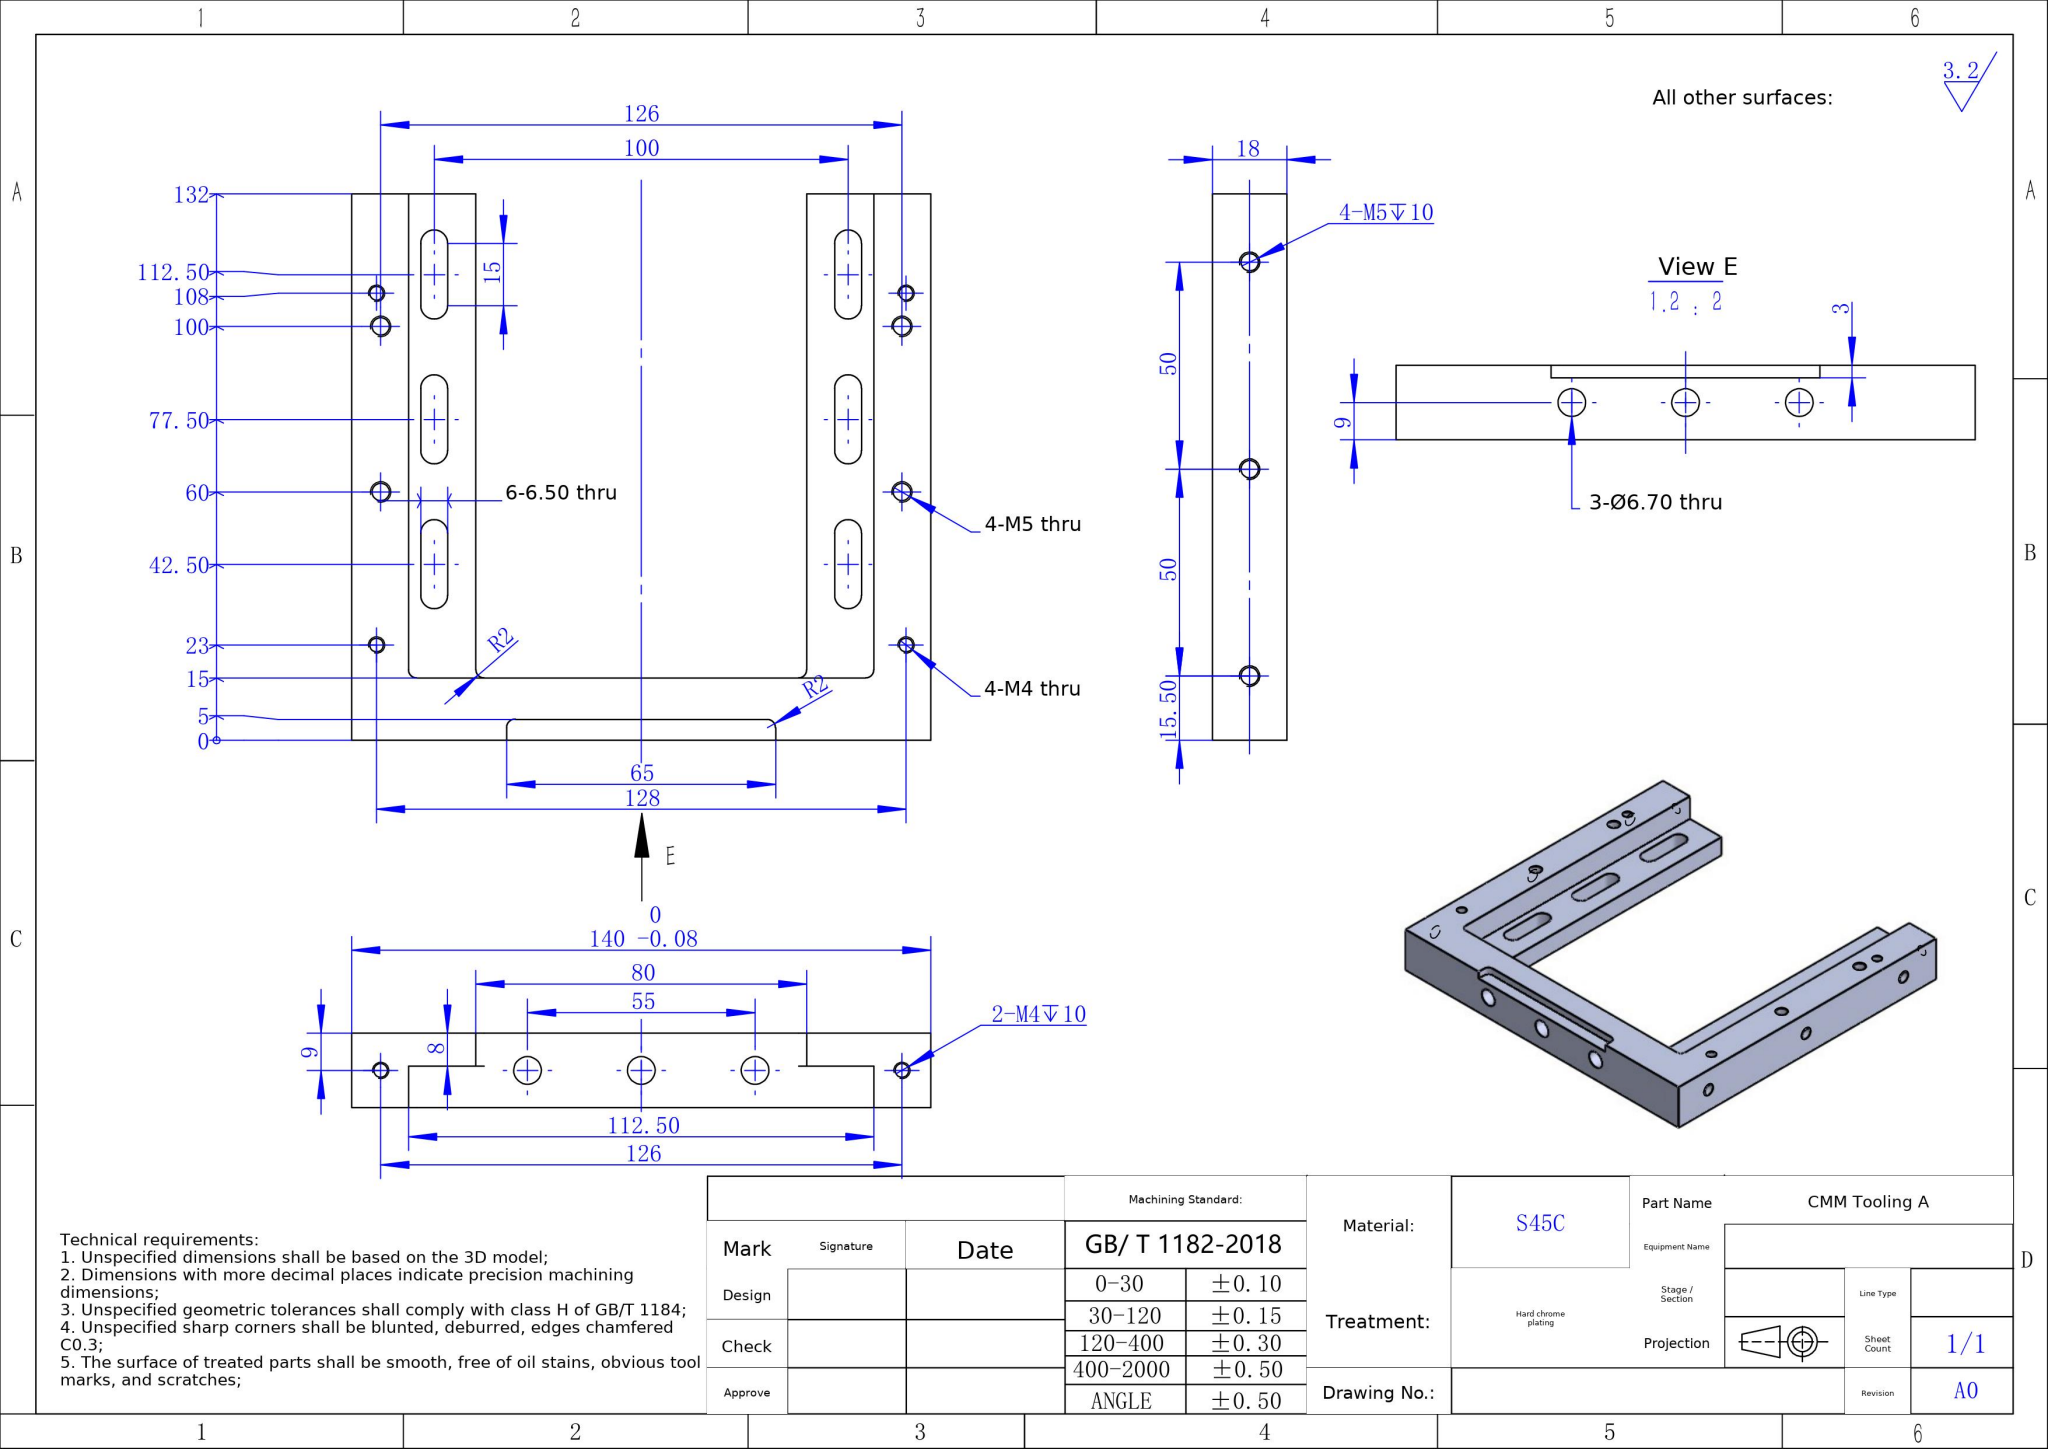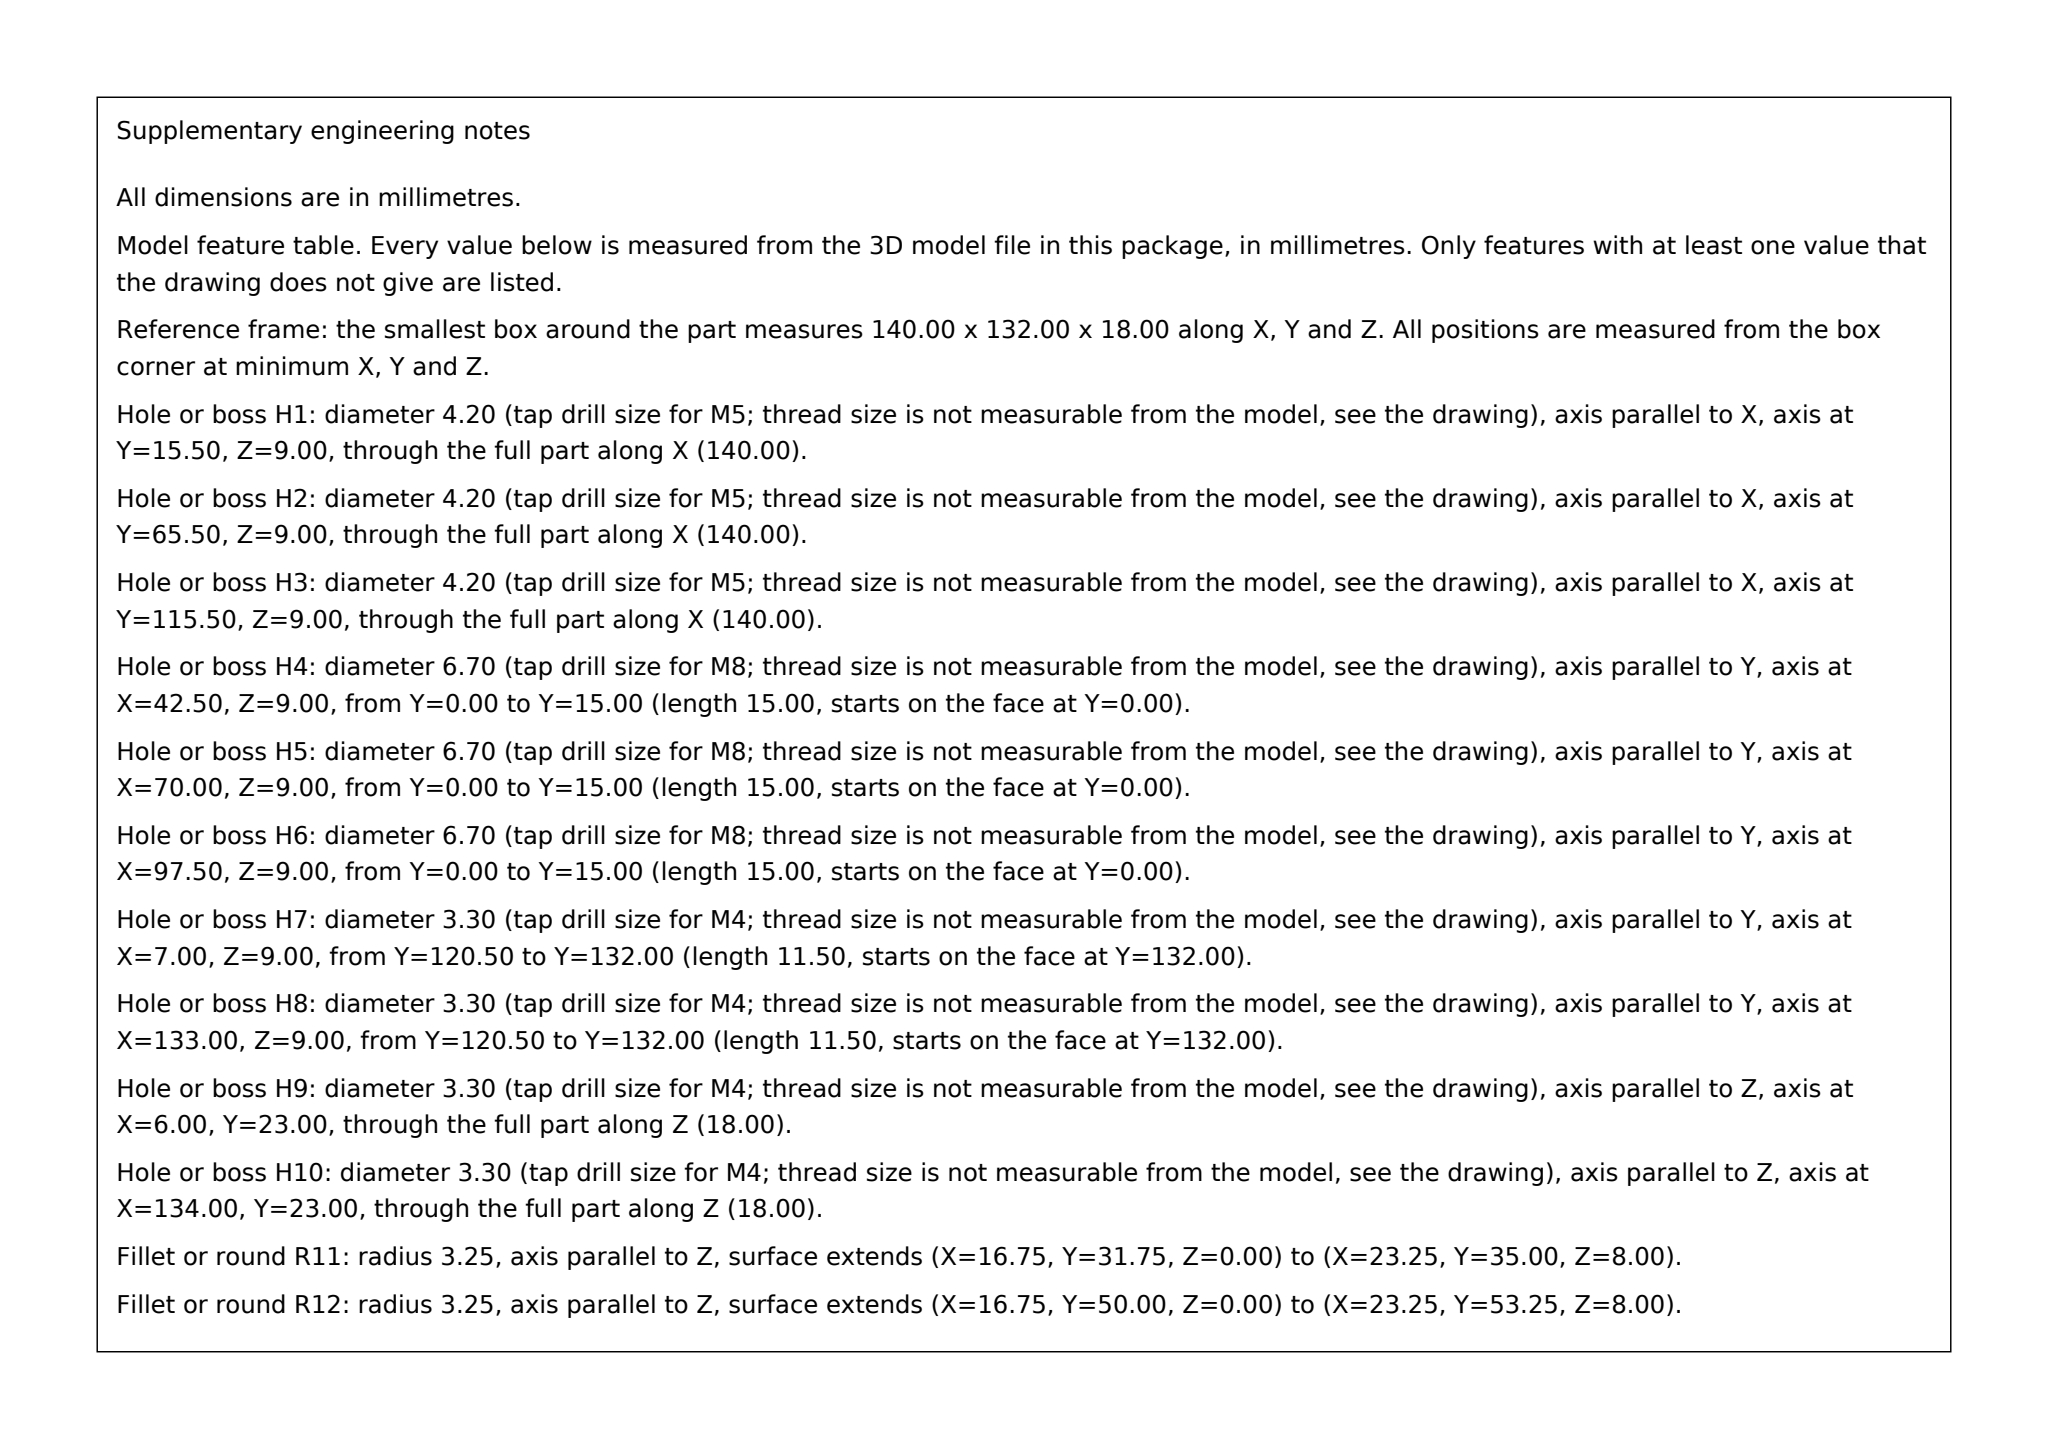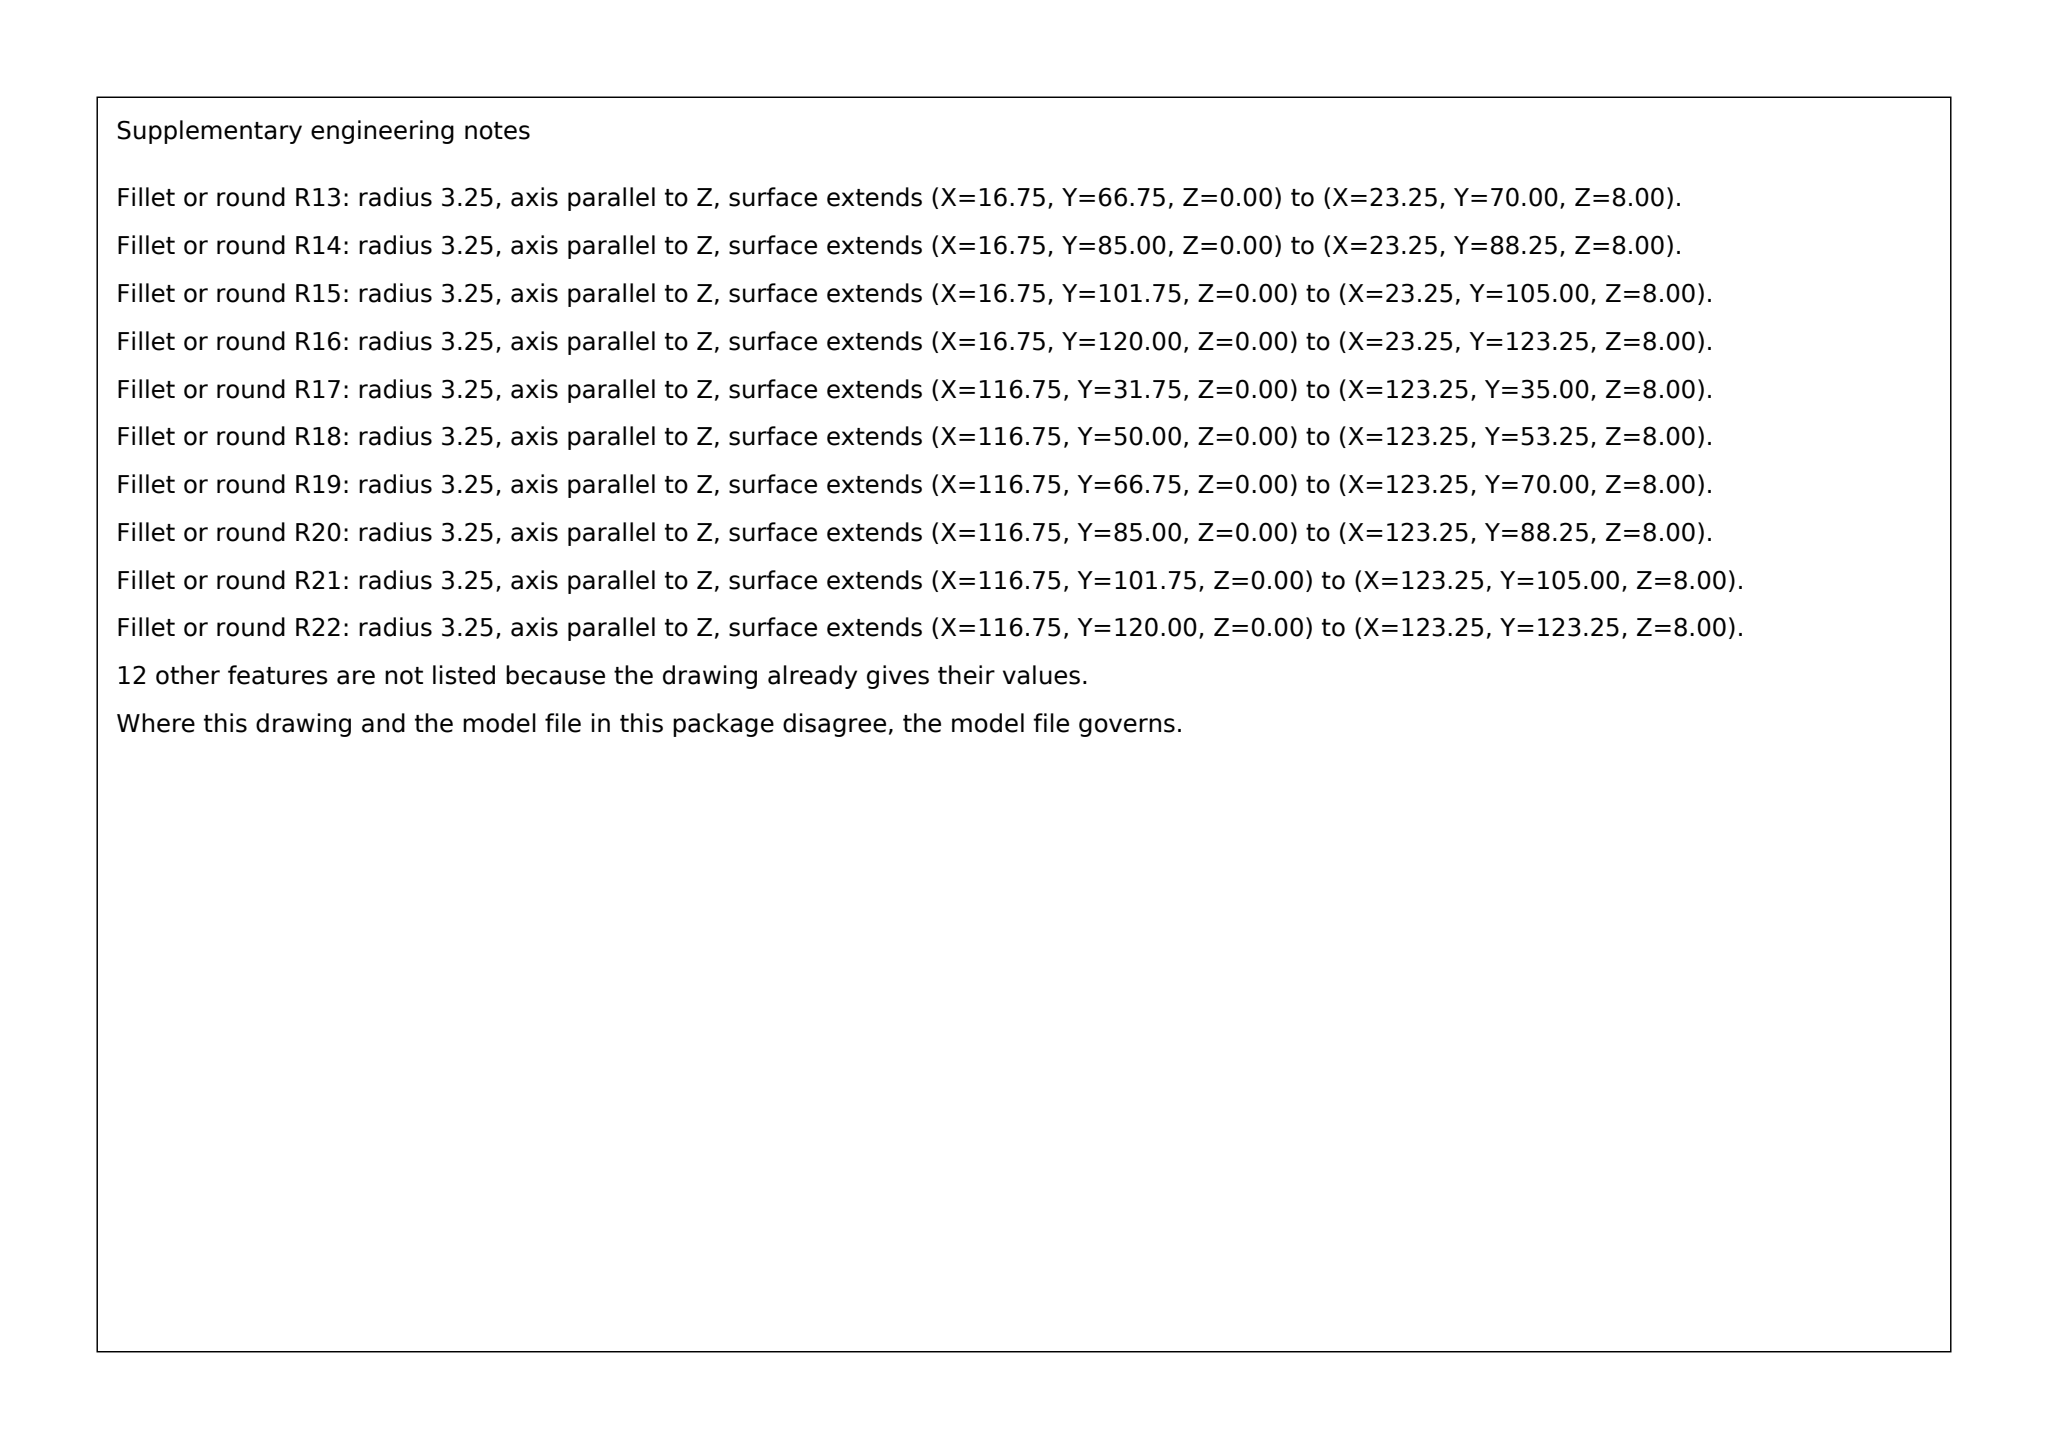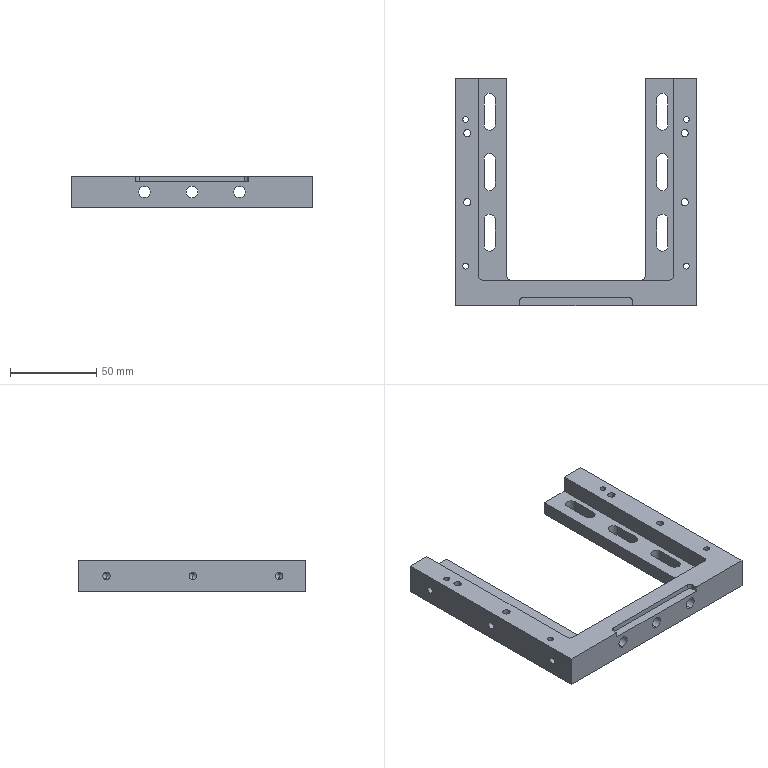Part | SolidWorks | mm | material S45C | 1 solid | 102 faces | box 140 x 132 x 18 mm | volume 114489 mm3 | cylinder 56 | plane 30 | cone 16 | commonest cylinder face diameters 4.2 x20 3.3 x12 6.5 x12 6.7 x6 4 x6